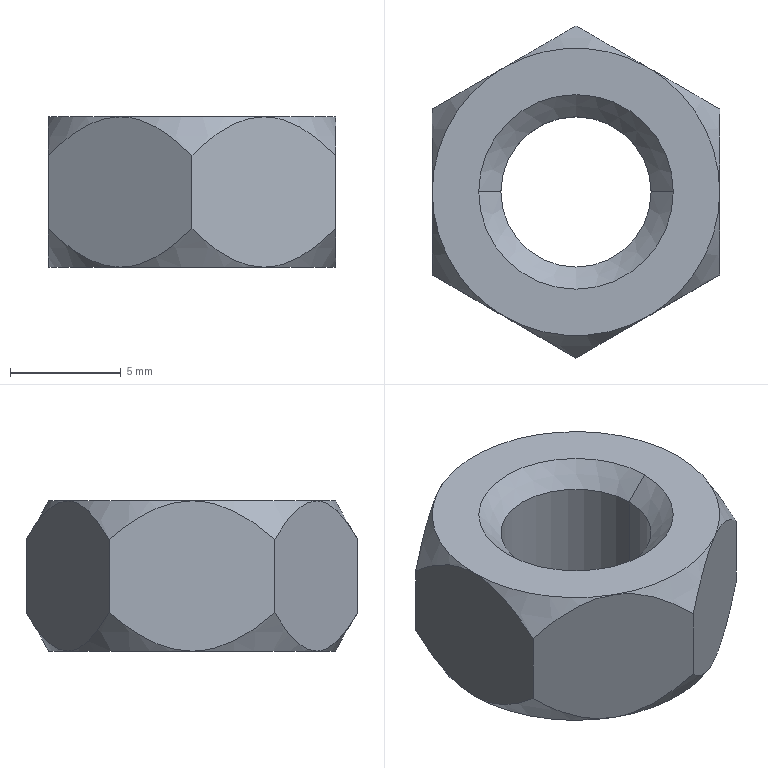Component | SolidWorks | Nut-3 | 1 solid | 26 faces | box 13 x 15.01 x 6.8 mm | volume 711 mm3 | cone 16 | plane 8 | cylinder 2 | commonest cylinder face diameters 6.8 x2
build123d program:
from build123d import *

# Parameters (mm, degrees)
BOSS_EXTRUDE1_DEPTH     = 3.4
SKETCH2_OUTSIDE_W       = 27.05
SKETCH2_OUTSIDE_H       = 29.062
SKETCH2_OUTSIDE_R       = 6.5
CUT_EXTRUDE1_DEPTH      = 6.8
CUT_EXTRUDE1_DRAFT      = -30
MIRROR1_COPY_1_SKETCH_W = 27.05
MIRROR1_COPY_1_SKETCH_H = 29.062
MIRROR1_COPY_1_SKETCH_R = 6.5
MIRROR1_COPY_1_DEPTH    = 6.8
MIRROR1_COPY_1_DRAFT    = -30
SKETCH5_W               = 3.4
SKETCH5_H               = 6.8
CHAMFER1_SIZE           = 1


with BuildPart() as part:
    # Sketch1 → Boss-Extrude1 (new, symmetric)
    with BuildSketch(Plane.XY):
        Polygon((0, 7.506), (-6.5, 3.753), (-6.5, -3.753), (0, -7.506), (6.5, -3.753), (6.5, 3.753), align=None)
    extrude(amount=BOSS_EXTRUDE1_DEPTH, both=True)


with BuildPart() as cut_extrude1_tool:
    # Sketch2 outside → Cut-Extrude1 (with draft: the straight prism first)
    with BuildSketch(Plane.XY.offset(3.4)):
        Rectangle(SKETCH2_OUTSIDE_W, SKETCH2_OUTSIDE_H)
        Circle(SKETCH2_OUTSIDE_R, mode=Mode.SUBTRACT)
    extrude(amount=-CUT_EXTRUDE1_DEPTH)
    # Cut-Extrude1: the draft: its side faces are tilted about the plane it starts from
    cut_extrude1_sides = [cut_extrude1_tool.faces().sort_by_distance(p)[0] for p in [
        (0, -14.531, 0),
        (13.525, 0, 0),
        (0, 14.531, 0),
        (-13.525, 0, 0),
        (-6.5, 0, 0),
    ]]
    draft(cut_extrude1_sides, Plane.XY.offset(3.4), CUT_EXTRUDE1_DRAFT)


with BuildPart() as part_1:
    add(part.part)

    # Cut-Extrude1: cut by cut_extrude1_tool
    add(cut_extrude1_tool.part, mode=Mode.SUBTRACT)


with BuildPart() as mirror1_copy_1_tool:
    # Mirror1 copy 1 sketch → Mirror1 copy 1 (with draft: the straight prism first)
    with BuildSketch(Plane(origin=(0, 0, -3.4), x_dir=(1, 0, 0), z_dir=(0, 0, -1))):
        Rectangle(MIRROR1_COPY_1_SKETCH_W, MIRROR1_COPY_1_SKETCH_H)
        Circle(MIRROR1_COPY_1_SKETCH_R, mode=Mode.SUBTRACT)
    extrude(amount=-MIRROR1_COPY_1_DEPTH)
    # Mirror1 copy 1: the draft: its side faces are tilted about the plane it starts from
    mirror1_copy_1_sides = [mirror1_copy_1_tool.faces().sort_by_distance(p)[0] for p in [
        (0, -14.531, 0),
        (13.525, 0, 0),
        (0, 14.531, 0),
        (-13.525, 0, 0),
        (-6.5, 0, 0),
    ]]
    draft(mirror1_copy_1_sides, Plane(origin=(0, 0, -3.4), x_dir=(1, 0, 0), z_dir=(0, 0, -1)), MIRROR1_COPY_1_DRAFT)


with BuildPart() as part_2:
    add(part_1.part)

    # Mirror1 copy 1: cut by mirror1_copy_1_tool
    add(mirror1_copy_1_tool.part, mode=Mode.SUBTRACT)

    # Sketch5 → M8 Tapped Hole1 (revolve, cut)
    with BuildSketch(Plane(origin=(0, 0, -3.4), x_dir=(0, 1, 0), z_dir=(1, 0, 0))):
        with Locations((1.7, 3.4)):
            Rectangle(SKETCH5_W, SKETCH5_H)
    revolve(axis=Axis((0, 0, -9.75), (0, 0, 1)), mode=Mode.SUBTRACT)

    # Chamfer1
    chamfer1_edges = [part_2.edges().sort_by_distance(p)[0] for p in [
        (0, -3.4, -3.4),
        (0, -3.4, 3.4),
    ]]
    chamfer(chamfer1_edges, length=CHAMFER1_SIZE)


solid = part_2.part

# Placed as in the assembly
solid = solid.moved(Location((-55.719, -28.485, 220.4), (0, 0, 0)))
STEP:
#1=CARTESIAN_POINT('',(-2.06,-1.121,8.583));
#2=VERTEX_POINT('',#1);
#3=CARTESIAN_POINT('',(-2.328,-1.121,8.583));
#4=VERTEX_POINT('',#3);
#5=CARTESIAN_POINT('',(-2.194,-1.121,8.583));
#6=DIRECTION('',(0.,0.,-1.));
#7=DIRECTION('',(-1.,0.,0.));
#8=AXIS2_PLACEMENT_3D('',#5,#6,#7);
#9=CIRCLE('',#8,0.1339);
#10=EDGE_CURVE('',#2,#4,#9,.T.);
#11=ORIENTED_EDGE('',*,*,#10,.F.);
#12=CARTESIAN_POINT('',(-2.02,-1.121,8.543));
#13=VERTEX_POINT('',#12);
#14=CARTESIAN_POINT('',(-2.02,-1.121,8.543));
#15=DIRECTION('',(0.7071,0.,-0.7071));
#16=VECTOR('',#15,39.37);
#17=LINE('',#14,#16);
#18=EDGE_CURVE('',#2,#13,#17,.T.);
#19=ORIENTED_EDGE('',*,*,#18,.T.);
#20=CARTESIAN_POINT('',(-2.367,-1.121,8.543));
#21=VERTEX_POINT('',#20);
#22=CARTESIAN_POINT('',(-2.194,-1.121,8.543));
#23=DIRECTION('',(0.,0.,1.));
#24=DIRECTION('',(-1.,0.,0.));
#25=AXIS2_PLACEMENT_3D('',#22,#23,#24);
#26=CIRCLE('',#25,0.1732);
#27=EDGE_CURVE('',#21,#13,#26,.T.);
#28=ORIENTED_EDGE('',*,*,#27,.F.);
#29=CARTESIAN_POINT('',(-2.367,-1.121,8.543));
#30=DIRECTION('',(-0.7071,0.,-0.7071));
#31=VECTOR('',#30,39.37);
#32=LINE('',#29,#31);
#33=EDGE_CURVE('',#4,#21,#32,.T.);
#34=ORIENTED_EDGE('',*,*,#33,.F.);
#35=EDGE_LOOP('',(#11,#19,#28,#34));
#36=FACE_OUTER_BOUND('',#35,.T.);
#37=CARTESIAN_POINT('',(-2.194,-1.121,8.543));
#38=DIRECTION('',(0.,0.,-1.));
#39=DIRECTION('',(-1.,0.,0.));
#40=AXIS2_PLACEMENT_3D('',#37,#38,#39);
#41=CONICAL_SURFACE('',#40,0.1732,0.7854);
#42=ADVANCED_FACE('',(#36),#41,.F.);
#43=CARTESIAN_POINT('',(-2.328,-1.121,8.772));
#44=VERTEX_POINT('',#43);
#45=CARTESIAN_POINT('',(-2.06,-1.121,8.772));
#46=VERTEX_POINT('',#45);
#47=CARTESIAN_POINT('',(-2.194,-1.121,8.772));
#48=DIRECTION('',(0.,0.,1.));
#49=DIRECTION('',(-1.,0.,0.));
#50=AXIS2_PLACEMENT_3D('',#47,#48,#49);
#51=CIRCLE('',#50,0.1339);
#52=EDGE_CURVE('',#44,#46,#51,.T.);
#53=ORIENTED_EDGE('',*,*,#52,.F.);
#54=CARTESIAN_POINT('',(-2.367,-1.121,8.811));
#55=VERTEX_POINT('',#54);
#56=CARTESIAN_POINT('',(-2.328,-1.121,8.772));
#57=DIRECTION('',(-0.7071,0.,0.7071));
#58=VECTOR('',#57,39.37);
#59=LINE('',#56,#58);
#60=EDGE_CURVE('',#44,#55,#59,.T.);
#61=ORIENTED_EDGE('',*,*,#60,.T.);
#62=CARTESIAN_POINT('',(-2.02,-1.121,8.811));
#63=VERTEX_POINT('',#62);
#64=CARTESIAN_POINT('',(-2.194,-1.121,8.811));
#65=DIRECTION('',(0.,0.,-1.));
#66=DIRECTION('',(-1.,0.,0.));
#67=AXIS2_PLACEMENT_3D('',#64,#65,#66);
#68=CIRCLE('',#67,0.1732);
#69=EDGE_CURVE('',#63,#55,#68,.T.);
#70=ORIENTED_EDGE('',*,*,#69,.F.);
#71=CARTESIAN_POINT('',(-2.06,-1.121,8.772));
#72=DIRECTION('',(0.7071,0.,0.7071));
#73=VECTOR('',#72,39.37);
#74=LINE('',#71,#73);
#75=EDGE_CURVE('',#46,#63,#74,.T.);
#76=ORIENTED_EDGE('',*,*,#75,.F.);
#77=EDGE_LOOP('',(#53,#61,#70,#76));
#78=FACE_OUTER_BOUND('',#77,.T.);
#79=CARTESIAN_POINT('',(-2.194,-1.121,8.772));
#80=DIRECTION('',(0.,0.,1.));
#81=DIRECTION('',(1.,0.,0.));
#82=AXIS2_PLACEMENT_3D('',#79,#80,#81);
#83=CONICAL_SURFACE('',#82,0.1339,0.7854);
#84=ADVANCED_FACE('',(#78),#83,.F.);
#85=ORIENTED_EDGE('',*,*,#10,.T.);
#86=CARTESIAN_POINT('',(-2.328,-1.121,8.811));
#87=DIRECTION('',(0.,0.,1.));
#88=VECTOR('',#87,39.37);
#89=LINE('',#86,#88);
#90=EDGE_CURVE('',#4,#44,#89,.T.);
#91=ORIENTED_EDGE('',*,*,#90,.T.);
#92=ORIENTED_EDGE('',*,*,#52,.T.);
#93=CARTESIAN_POINT('',(-2.06,-1.121,8.811));
#94=DIRECTION('',(0.,0.,1.));
#95=VECTOR('',#94,39.37);
#96=LINE('',#93,#95);
#97=EDGE_CURVE('',#2,#46,#96,.T.);
#98=ORIENTED_EDGE('',*,*,#97,.F.);
#99=EDGE_LOOP('',(#85,#91,#92,#98));
#100=FACE_OUTER_BOUND('',#99,.T.);
#101=CARTESIAN_POINT('',(-2.194,-1.121,8.811));
#102=DIRECTION('',(0.,0.,1.));
#103=DIRECTION('',(1.,0.,0.));
#104=AXIS2_PLACEMENT_3D('',#101,#102,#103);
#105=CYLINDRICAL_SURFACE('',#104,0.1339);
#106=ADVANCED_FACE('',(#100),#105,.F.);
#107=CARTESIAN_POINT('',(-2.45,-0.9737,8.612));
#108=VERTEX_POINT('',#107);
#109=CARTESIAN_POINT('',(-2.45,-0.9737,8.742));
#110=VERTEX_POINT('',#109);
#111=CARTESIAN_POINT('',(-2.45,-0.9737,8.543));
#112=DIRECTION('',(0.,0.,1.));
#113=VECTOR('',#112,39.37);
#114=LINE('',#111,#113);
#115=EDGE_CURVE('',#108,#110,#114,.T.);
#116=ORIENTED_EDGE('',*,*,#115,.T.);
#117=CARTESIAN_POINT('',(-2.322,-0.8998,8.811));
#118=VERTEX_POINT('',#117);
#119=CARTESIAN_POINT('',(-2.45,-0.9737,8.742));
#120=CARTESIAN_POINT('',(-2.44,-0.9685,8.752));
#121=CARTESIAN_POINT('',(-2.431,-0.9631,8.76));
#122=CARTESIAN_POINT('',(-2.412,-0.9518,8.776));
#123=CARTESIAN_POINT('',(-2.402,-0.946,8.784));
#124=CARTESIAN_POINT('',(-2.38,-0.9337,8.796));
#125=CARTESIAN_POINT('',(-2.369,-0.9271,8.802));
#126=CARTESIAN_POINT('',(-2.352,-0.9171,8.807));
#127=CARTESIAN_POINT('',(-2.346,-0.9137,8.809));
#128=CARTESIAN_POINT('',(-2.334,-0.9068,8.811));
#129=CARTESIAN_POINT('',(-2.328,-0.9033,8.811));
#130=CARTESIAN_POINT('',(-2.322,-0.8998,8.811));
#131=B_SPLINE_CURVE_WITH_KNOTS('',3,(#119,#120,#121,#122,#123,#124,#125,#126,#127,#128,#129,#130),.UNSPECIFIED.,.F.,.F.,(4,2,2,2,2,4),(0.0000003,0.001051,0.002101,0.003151,0.003676,0.004201),.UNSPECIFIED.);
#132=EDGE_CURVE('',#110,#118,#131,.T.);
#133=ORIENTED_EDGE('',*,*,#132,.T.);
#134=CARTESIAN_POINT('',(-2.194,-0.826,8.742));
#135=VERTEX_POINT('',#134);
#136=CARTESIAN_POINT('',(-2.322,-0.8998,8.811));
#137=CARTESIAN_POINT('',(-2.31,-0.8929,8.811));
#138=CARTESIAN_POINT('',(-2.298,-0.8861,8.809));
#139=CARTESIAN_POINT('',(-2.274,-0.8726,8.802));
#140=CARTESIAN_POINT('',(-2.263,-0.8662,8.796));
#141=CARTESIAN_POINT('',(-2.242,-0.8539,8.784));
#142=CARTESIAN_POINT('',(-2.232,-0.848,8.776));
#143=CARTESIAN_POINT('',(-2.212,-0.8367,8.76));
#144=CARTESIAN_POINT('',(-2.203,-0.8312,8.752));
#145=CARTESIAN_POINT('',(-2.194,-0.826,8.742));
#146=B_SPLINE_CURVE_WITH_KNOTS('',3,(#136,#137,#138,#139,#140,#141,#142,#143,#144,#145),.UNSPECIFIED.,.F.,.F.,(4,2,2,2,4),(0.004201,0.00525,0.006298,0.007347,0.008395),.UNSPECIFIED.);
#147=EDGE_CURVE('',#118,#135,#146,.T.);
#148=ORIENTED_EDGE('',*,*,#147,.T.);
#149=CARTESIAN_POINT('',(-2.194,-0.826,8.612));
#150=VERTEX_POINT('',#149);
#151=CARTESIAN_POINT('',(-2.194,-0.826,8.543));
#152=DIRECTION('',(0.,0.,1.));
#153=VECTOR('',#152,39.37);
#154=LINE('',#151,#153);
#155=EDGE_CURVE('',#150,#135,#154,.T.);
#156=ORIENTED_EDGE('',*,*,#155,.F.);
#157=CARTESIAN_POINT('',(-2.322,-0.8998,8.543));
#158=VERTEX_POINT('',#157);
#159=CARTESIAN_POINT('',(-2.322,-0.8998,8.543));
#160=CARTESIAN_POINT('',(-2.31,-0.8929,8.543));
#161=CARTESIAN_POINT('',(-2.298,-0.8861,8.545));
#162=CARTESIAN_POINT('',(-2.274,-0.8726,8.553));
#163=CARTESIAN_POINT('',(-2.263,-0.8662,8.558));
#164=CARTESIAN_POINT('',(-2.242,-0.8539,8.571));
#165=CARTESIAN_POINT('',(-2.232,-0.848,8.578));
#166=CARTESIAN_POINT('',(-2.212,-0.8367,8.594));
#167=CARTESIAN_POINT('',(-2.203,-0.8312,8.603));
#168=CARTESIAN_POINT('',(-2.194,-0.826,8.612));
#169=B_SPLINE_CURVE_WITH_KNOTS('',3,(#159,#160,#161,#162,#163,#164,#165,#166,#167,#168),.UNSPECIFIED.,.F.,.F.,(4,2,2,2,4),(0.004201,0.00525,0.006298,0.007347,0.008395),.UNSPECIFIED.);
#170=EDGE_CURVE('',#158,#150,#169,.T.);
#171=ORIENTED_EDGE('',*,*,#170,.F.);
#172=CARTESIAN_POINT('',(-2.45,-0.9737,8.612));
#173=CARTESIAN_POINT('',(-2.44,-0.9685,8.603));
#174=CARTESIAN_POINT('',(-2.431,-0.9631,8.594));
#175=CARTESIAN_POINT('',(-2.412,-0.9518,8.578));
#176=CARTESIAN_POINT('',(-2.402,-0.946,8.571));
#177=CARTESIAN_POINT('',(-2.38,-0.9337,8.558));
#178=CARTESIAN_POINT('',(-2.369,-0.9271,8.553));
#179=CARTESIAN_POINT('',(-2.352,-0.9171,8.547));
#180=CARTESIAN_POINT('',(-2.346,-0.9137,8.546));
#181=CARTESIAN_POINT('',(-2.334,-0.9068,8.544));
#182=CARTESIAN_POINT('',(-2.328,-0.9033,8.543));
#183=CARTESIAN_POINT('',(-2.322,-0.8998,8.543));
#184=B_SPLINE_CURVE_WITH_KNOTS('',3,(#172,#173,#174,#175,#176,#177,#178,#179,#180,#181,#182,#183),.UNSPECIFIED.,.F.,.F.,(4,2,2,2,2,4),(0.0000003,0.001051,0.002101,0.003151,0.003676,0.004201),.UNSPECIFIED.);
#185=EDGE_CURVE('',#108,#158,#184,.T.);
#186=ORIENTED_EDGE('',*,*,#185,.F.);
#187=EDGE_LOOP('',(#116,#133,#148,#156,#171,#186));
#188=FACE_OUTER_BOUND('',#187,.T.);
#189=CARTESIAN_POINT('',(-2.45,-0.9737,8.543));
#190=DIRECTION('',(0.5,-0.866,0.));
#191=DIRECTION('',(-0.866,-0.5,0.));
#192=AXIS2_PLACEMENT_3D('',#189,#190,#191);
#193=PLANE('',#192);
#194=ADVANCED_FACE('',(#188),#193,.F.);
#195=ORIENTED_EDGE('',*,*,#155,.T.);
#196=CARTESIAN_POINT('',(-2.066,-0.8998,8.811));
#197=VERTEX_POINT('',#196);
#198=CARTESIAN_POINT('',(-2.194,-0.826,8.742));
#199=CARTESIAN_POINT('',(-2.185,-0.8312,8.752));
#200=CARTESIAN_POINT('',(-2.175,-0.8366,8.76));
#201=CARTESIAN_POINT('',(-2.156,-0.8479,8.776));
#202=CARTESIAN_POINT('',(-2.146,-0.8537,8.784));
#203=CARTESIAN_POINT('',(-2.124,-0.866,8.796));
#204=CARTESIAN_POINT('',(-2.113,-0.8725,8.802));
#205=CARTESIAN_POINT('',(-2.096,-0.8826,8.807));
#206=CARTESIAN_POINT('',(-2.09,-0.886,8.809));
#207=CARTESIAN_POINT('',(-2.078,-0.8929,8.811));
#208=CARTESIAN_POINT('',(-2.072,-0.8964,8.811));
#209=CARTESIAN_POINT('',(-2.066,-0.8998,8.811));
#210=B_SPLINE_CURVE_WITH_KNOTS('',3,(#198,#199,#200,#201,#202,#203,#204,#205,#206,#207,#208,#209),.UNSPECIFIED.,.F.,.F.,(4,2,2,2,2,4),(0.0000003,0.001051,0.002101,0.003151,0.003676,0.004201),.UNSPECIFIED.);
#211=EDGE_CURVE('',#135,#197,#210,.T.);
#212=ORIENTED_EDGE('',*,*,#211,.T.);
#213=CARTESIAN_POINT('',(-1.938,-0.9737,8.742));
#214=VERTEX_POINT('',#213);
#215=CARTESIAN_POINT('',(-2.066,-0.8998,8.811));
#216=CARTESIAN_POINT('',(-2.054,-0.9068,8.811));
#217=CARTESIAN_POINT('',(-2.042,-0.9136,8.809));
#218=CARTESIAN_POINT('',(-2.019,-0.9271,8.802));
#219=CARTESIAN_POINT('',(-2.007,-0.9335,8.796));
#220=CARTESIAN_POINT('',(-1.986,-0.9458,8.784));
#221=CARTESIAN_POINT('',(-1.976,-0.9517,8.776));
#222=CARTESIAN_POINT('',(-1.956,-0.963,8.76));
#223=CARTESIAN_POINT('',(-1.947,-0.9685,8.752));
#224=CARTESIAN_POINT('',(-1.938,-0.9737,8.742));
#225=B_SPLINE_CURVE_WITH_KNOTS('',3,(#215,#216,#217,#218,#219,#220,#221,#222,#223,#224),.UNSPECIFIED.,.F.,.F.,(4,2,2,2,4),(0.004201,0.00525,0.006298,0.007347,0.008395),.UNSPECIFIED.);
#226=EDGE_CURVE('',#197,#214,#225,.T.);
#227=ORIENTED_EDGE('',*,*,#226,.T.);
#228=CARTESIAN_POINT('',(-1.938,-0.9737,8.612));
#229=VERTEX_POINT('',#228);
#230=CARTESIAN_POINT('',(-1.938,-0.9737,8.543));
#231=DIRECTION('',(0.,0.,1.));
#232=VECTOR('',#231,39.37);
#233=LINE('',#230,#232);
#234=EDGE_CURVE('',#229,#214,#233,.T.);
#235=ORIENTED_EDGE('',*,*,#234,.F.);
#236=CARTESIAN_POINT('',(-2.066,-0.8998,8.543));
#237=VERTEX_POINT('',#236);
#238=CARTESIAN_POINT('',(-2.066,-0.8998,8.543));
#239=CARTESIAN_POINT('',(-2.054,-0.9068,8.543));
#240=CARTESIAN_POINT('',(-2.042,-0.9136,8.545));
#241=CARTESIAN_POINT('',(-2.019,-0.9271,8.553));
#242=CARTESIAN_POINT('',(-2.007,-0.9335,8.558));
#243=CARTESIAN_POINT('',(-1.986,-0.9458,8.571));
#244=CARTESIAN_POINT('',(-1.976,-0.9517,8.578));
#245=CARTESIAN_POINT('',(-1.956,-0.963,8.594));
#246=CARTESIAN_POINT('',(-1.947,-0.9685,8.603));
#247=CARTESIAN_POINT('',(-1.938,-0.9737,8.612));
#248=B_SPLINE_CURVE_WITH_KNOTS('',3,(#238,#239,#240,#241,#242,#243,#244,#245,#246,#247),.UNSPECIFIED.,.F.,.F.,(4,2,2,2,4),(0.004201,0.00525,0.006298,0.007347,0.008395),.UNSPECIFIED.);
#249=EDGE_CURVE('',#237,#229,#248,.T.);
#250=ORIENTED_EDGE('',*,*,#249,.F.);
#251=CARTESIAN_POINT('',(-2.194,-0.826,8.612));
#252=CARTESIAN_POINT('',(-2.185,-0.8312,8.603));
#253=CARTESIAN_POINT('',(-2.175,-0.8366,8.594));
#254=CARTESIAN_POINT('',(-2.156,-0.8479,8.578));
#255=CARTESIAN_POINT('',(-2.146,-0.8537,8.571));
#256=CARTESIAN_POINT('',(-2.124,-0.866,8.558));
#257=CARTESIAN_POINT('',(-2.113,-0.8725,8.553));
#258=CARTESIAN_POINT('',(-2.096,-0.8826,8.547));
#259=CARTESIAN_POINT('',(-2.09,-0.886,8.546));
#260=CARTESIAN_POINT('',(-2.078,-0.8929,8.544));
#261=CARTESIAN_POINT('',(-2.072,-0.8964,8.543));
#262=CARTESIAN_POINT('',(-2.066,-0.8998,8.543));
#263=B_SPLINE_CURVE_WITH_KNOTS('',3,(#251,#252,#253,#254,#255,#256,#257,#258,#259,#260,#261,#262),.UNSPECIFIED.,.F.,.F.,(4,2,2,2,2,4),(0.0000003,0.001051,0.002101,0.003151,0.003676,0.004201),.UNSPECIFIED.);
#264=EDGE_CURVE('',#150,#237,#263,.T.);
#265=ORIENTED_EDGE('',*,*,#264,.F.);
#266=EDGE_LOOP('',(#195,#212,#227,#235,#250,#265));
#267=FACE_OUTER_BOUND('',#266,.T.);
#268=CARTESIAN_POINT('',(-2.194,-0.826,8.543));
#269=DIRECTION('',(-0.5,-0.866,0.));
#270=DIRECTION('',(-0.866,0.5,0.));
#271=AXIS2_PLACEMENT_3D('',#268,#269,#270);
#272=PLANE('',#271);
#273=ADVANCED_FACE('',(#267),#272,.F.);
#274=ORIENTED_EDGE('',*,*,#234,.T.);
#275=CARTESIAN_POINT('',(-1.938,-1.121,8.811));
#276=VERTEX_POINT('',#275);
#277=CARTESIAN_POINT('',(-1.938,-0.9737,8.742));
#278=CARTESIAN_POINT('',(-1.938,-0.9841,8.751));
#279=CARTESIAN_POINT('',(-1.938,-0.9948,8.76));
#280=CARTESIAN_POINT('',(-1.938,-1.017,8.776));
#281=CARTESIAN_POINT('',(-1.938,-1.029,8.783));
#282=CARTESIAN_POINT('',(-1.938,-1.053,8.796));
#283=CARTESIAN_POINT('',(-1.938,-1.067,8.802));
#284=CARTESIAN_POINT('',(-1.938,-1.087,8.807));
#285=CARTESIAN_POINT('',(-1.938,-1.094,8.809));
#286=CARTESIAN_POINT('',(-1.938,-1.107,8.811));
#287=CARTESIAN_POINT('',(-1.938,-1.114,8.811));
#288=CARTESIAN_POINT('',(-1.938,-1.121,8.811));
#289=B_SPLINE_CURVE_WITH_KNOTS('',3,(#277,#278,#279,#280,#281,#282,#283,#284,#285,#286,#287,#288),.UNSPECIFIED.,.F.,.F.,(4,2,2,2,2,4),(0.01696,0.01802,0.01907,0.02012,0.02065,0.02117),.UNSPECIFIED.);
#290=EDGE_CURVE('',#214,#276,#289,.T.);
#291=ORIENTED_EDGE('',*,*,#290,.T.);
#292=CARTESIAN_POINT('',(-1.938,-1.269,8.742));
#293=VERTEX_POINT('',#292);
#294=CARTESIAN_POINT('',(-1.938,-1.121,8.811));
#295=CARTESIAN_POINT('',(-1.938,-1.135,8.811));
#296=CARTESIAN_POINT('',(-1.938,-1.149,8.809));
#297=CARTESIAN_POINT('',(-1.938,-1.169,8.804));
#298=CARTESIAN_POINT('',(-1.938,-1.176,8.801));
#299=CARTESIAN_POINT('',(-1.938,-1.189,8.796));
#300=CARTESIAN_POINT('',(-1.938,-1.195,8.793));
#301=CARTESIAN_POINT('',(-1.938,-1.226,8.777));
#302=CARTESIAN_POINT('',(-1.938,-1.248,8.761));
#303=CARTESIAN_POINT('',(-1.938,-1.269,8.742));
#304=B_SPLINE_CURVE_WITH_KNOTS('',3,(#294,#295,#296,#297,#298,#299,#300,#301,#302,#303),.UNSPECIFIED.,.F.,.F.,(4,2,2,2,4),(0.02117,0.02222,0.02274,0.02326,0.02535),.UNSPECIFIED.);
#305=EDGE_CURVE('',#276,#293,#304,.T.);
#306=ORIENTED_EDGE('',*,*,#305,.T.);
#307=CARTESIAN_POINT('',(-1.938,-1.269,8.612));
#308=VERTEX_POINT('',#307);
#309=CARTESIAN_POINT('',(-1.938,-1.269,8.543));
#310=DIRECTION('',(0.,0.,1.));
#311=VECTOR('',#310,39.37);
#312=LINE('',#309,#311);
#313=EDGE_CURVE('',#308,#293,#312,.T.);
#314=ORIENTED_EDGE('',*,*,#313,.F.);
#315=CARTESIAN_POINT('',(-1.938,-1.121,8.543));
#316=VERTEX_POINT('',#315);
#317=CARTESIAN_POINT('',(-1.938,-1.121,8.543));
#318=CARTESIAN_POINT('',(-1.938,-1.135,8.543));
#319=CARTESIAN_POINT('',(-1.938,-1.149,8.545));
#320=CARTESIAN_POINT('',(-1.938,-1.169,8.551));
#321=CARTESIAN_POINT('',(-1.938,-1.176,8.553));
#322=CARTESIAN_POINT('',(-1.938,-1.189,8.558));
#323=CARTESIAN_POINT('',(-1.938,-1.195,8.561));
#324=CARTESIAN_POINT('',(-1.938,-1.226,8.577));
#325=CARTESIAN_POINT('',(-1.938,-1.248,8.594));
#326=CARTESIAN_POINT('',(-1.938,-1.269,8.612));
#327=B_SPLINE_CURVE_WITH_KNOTS('',3,(#317,#318,#319,#320,#321,#322,#323,#324,#325,#326),.UNSPECIFIED.,.F.,.F.,(4,2,2,2,4),(0.02117,0.02222,0.02274,0.02326,0.02535),.UNSPECIFIED.);
#328=EDGE_CURVE('',#316,#308,#327,.T.);
#329=ORIENTED_EDGE('',*,*,#328,.F.);
#330=CARTESIAN_POINT('',(-1.938,-0.9737,8.612));
#331=CARTESIAN_POINT('',(-1.938,-0.9841,8.603));
#332=CARTESIAN_POINT('',(-1.938,-0.9948,8.594));
#333=CARTESIAN_POINT('',(-1.938,-1.017,8.578));
#334=CARTESIAN_POINT('',(-1.938,-1.029,8.571));
#335=CARTESIAN_POINT('',(-1.938,-1.053,8.558));
#336=CARTESIAN_POINT('',(-1.938,-1.067,8.553));
#337=CARTESIAN_POINT('',(-1.938,-1.087,8.547));
#338=CARTESIAN_POINT('',(-1.938,-1.094,8.546));
#339=CARTESIAN_POINT('',(-1.938,-1.107,8.544));
#340=CARTESIAN_POINT('',(-1.938,-1.114,8.543));
#341=CARTESIAN_POINT('',(-1.938,-1.121,8.543));
#342=B_SPLINE_CURVE_WITH_KNOTS('',3,(#330,#331,#332,#333,#334,#335,#336,#337,#338,#339,#340,#341),.UNSPECIFIED.,.F.,.F.,(4,2,2,2,2,4),(0.01696,0.01802,0.01907,0.02012,0.02065,0.02117),.UNSPECIFIED.);
#343=EDGE_CURVE('',#229,#316,#342,.T.);
#344=ORIENTED_EDGE('',*,*,#343,.F.);
#345=EDGE_LOOP('',(#274,#291,#306,#314,#329,#344));
#346=FACE_OUTER_BOUND('',#345,.T.);
#347=CARTESIAN_POINT('',(-1.938,-0.9737,8.543));
#348=DIRECTION('',(-1.,0.,0.));
#349=DIRECTION('',(0.,1.,0.));
#350=AXIS2_PLACEMENT_3D('',#347,#348,#349);
#351=PLANE('',#350);
#352=ADVANCED_FACE('',(#346),#351,.F.);
#353=ORIENTED_EDGE('',*,*,#313,.T.);
#354=CARTESIAN_POINT('',(-2.066,-1.343,8.811));
#355=VERTEX_POINT('',#354);
#356=CARTESIAN_POINT('',(-1.938,-1.269,8.742));
#357=CARTESIAN_POINT('',(-1.947,-1.274,8.752));
#358=CARTESIAN_POINT('',(-1.956,-1.28,8.76));
#359=CARTESIAN_POINT('',(-1.976,-1.291,8.776));
#360=CARTESIAN_POINT('',(-1.986,-1.297,8.784));
#361=CARTESIAN_POINT('',(-2.007,-1.309,8.796));
#362=CARTESIAN_POINT('',(-2.018,-1.316,8.802));
#363=CARTESIAN_POINT('',(-2.036,-1.326,8.807));
#364=CARTESIAN_POINT('',(-2.042,-1.329,8.809));
#365=CARTESIAN_POINT('',(-2.054,-1.336,8.811));
#366=CARTESIAN_POINT('',(-2.06,-1.34,8.811));
#367=CARTESIAN_POINT('',(-2.066,-1.343,8.811));
#368=B_SPLINE_CURVE_WITH_KNOTS('',3,(#356,#357,#358,#359,#360,#361,#362,#363,#364,#365,#366,#367),.UNSPECIFIED.,.F.,.F.,(4,2,2,2,2,4),(0.0000003,0.001051,0.002101,0.003151,0.003676,0.004201),.UNSPECIFIED.);
#369=EDGE_CURVE('',#293,#355,#368,.T.);
#370=ORIENTED_EDGE('',*,*,#369,.T.);
#371=CARTESIAN_POINT('',(-2.194,-1.417,8.742));
#372=VERTEX_POINT('',#371);
#373=CARTESIAN_POINT('',(-2.066,-1.343,8.811));
#374=CARTESIAN_POINT('',(-2.078,-1.35,8.811));
#375=CARTESIAN_POINT('',(-2.09,-1.357,8.809));
#376=CARTESIAN_POINT('',(-2.113,-1.37,8.802));
#377=CARTESIAN_POINT('',(-2.124,-1.377,8.796));
#378=CARTESIAN_POINT('',(-2.145,-1.389,8.784));
#379=CARTESIAN_POINT('',(-2.155,-1.395,8.776));
#380=CARTESIAN_POINT('',(-2.175,-1.406,8.76));
#381=CARTESIAN_POINT('',(-2.185,-1.412,8.752));
#382=CARTESIAN_POINT('',(-2.194,-1.417,8.742));
#383=B_SPLINE_CURVE_WITH_KNOTS('',3,(#373,#374,#375,#376,#377,#378,#379,#380,#381,#382),.UNSPECIFIED.,.F.,.F.,(4,2,2,2,4),(0.004201,0.00525,0.006298,0.007347,0.008395),.UNSPECIFIED.);
#384=EDGE_CURVE('',#355,#372,#383,.T.);
#385=ORIENTED_EDGE('',*,*,#384,.T.);
#386=CARTESIAN_POINT('',(-2.194,-1.417,8.612));
#387=VERTEX_POINT('',#386);
#388=CARTESIAN_POINT('',(-2.194,-1.417,8.543));
#389=DIRECTION('',(0.,0.,1.));
#390=VECTOR('',#389,39.37);
#391=LINE('',#388,#390);
#392=EDGE_CURVE('',#387,#372,#391,.T.);
#393=ORIENTED_EDGE('',*,*,#392,.F.);
#394=CARTESIAN_POINT('',(-2.066,-1.343,8.543));
#395=VERTEX_POINT('',#394);
#396=CARTESIAN_POINT('',(-2.066,-1.343,8.543));
#397=CARTESIAN_POINT('',(-2.078,-1.35,8.543));
#398=CARTESIAN_POINT('',(-2.09,-1.357,8.545));
#399=CARTESIAN_POINT('',(-2.113,-1.37,8.553));
#400=CARTESIAN_POINT('',(-2.124,-1.377,8.558));
#401=CARTESIAN_POINT('',(-2.145,-1.389,8.571));
#402=CARTESIAN_POINT('',(-2.155,-1.395,8.578));
#403=CARTESIAN_POINT('',(-2.175,-1.406,8.594));
#404=CARTESIAN_POINT('',(-2.185,-1.412,8.603));
#405=CARTESIAN_POINT('',(-2.194,-1.417,8.612));
#406=B_SPLINE_CURVE_WITH_KNOTS('',3,(#396,#397,#398,#399,#400,#401,#402,#403,#404,#405),.UNSPECIFIED.,.F.,.F.,(4,2,2,2,4),(0.004201,0.00525,0.006298,0.007347,0.008395),.UNSPECIFIED.);
#407=EDGE_CURVE('',#395,#387,#406,.T.);
#408=ORIENTED_EDGE('',*,*,#407,.F.);
#409=CARTESIAN_POINT('',(-1.938,-1.269,8.612));
#410=CARTESIAN_POINT('',(-1.947,-1.274,8.603));
#411=CARTESIAN_POINT('',(-1.956,-1.28,8.594));
#412=CARTESIAN_POINT('',(-1.976,-1.291,8.578));
#413=CARTESIAN_POINT('',(-1.986,-1.297,8.571));
#414=CARTESIAN_POINT('',(-2.007,-1.309,8.558));
#415=CARTESIAN_POINT('',(-2.018,-1.316,8.553));
#416=CARTESIAN_POINT('',(-2.036,-1.326,8.547));
#417=CARTESIAN_POINT('',(-2.042,-1.329,8.546));
#418=CARTESIAN_POINT('',(-2.054,-1.336,8.544));
#419=CARTESIAN_POINT('',(-2.06,-1.34,8.543));
#420=CARTESIAN_POINT('',(-2.066,-1.343,8.543));
#421=B_SPLINE_CURVE_WITH_KNOTS('',3,(#409,#410,#411,#412,#413,#414,#415,#416,#417,#418,#419,#420),.UNSPECIFIED.,.F.,.F.,(4,2,2,2,2,4),(0.0000003,0.001051,0.002101,0.003151,0.003676,0.004201),.UNSPECIFIED.);
#422=EDGE_CURVE('',#308,#395,#421,.T.);
#423=ORIENTED_EDGE('',*,*,#422,.F.);
#424=EDGE_LOOP('',(#353,#370,#385,#393,#408,#423));
#425=FACE_OUTER_BOUND('',#424,.T.);
#426=CARTESIAN_POINT('',(-1.938,-1.269,8.543));
#427=DIRECTION('',(-0.5,0.866,0.));
#428=DIRECTION('',(0.866,0.5,0.));
#429=AXIS2_PLACEMENT_3D('',#426,#427,#428);
#430=PLANE('',#429);
#431=ADVANCED_FACE('',(#425),#430,.F.);
#432=ORIENTED_EDGE('',*,*,#392,.T.);
#433=CARTESIAN_POINT('',(-2.322,-1.343,8.811));
#434=VERTEX_POINT('',#433);
#435=CARTESIAN_POINT('',(-2.194,-1.417,8.742));
#436=CARTESIAN_POINT('',(-2.203,-1.412,8.752));
#437=CARTESIAN_POINT('',(-2.212,-1.406,8.76));
#438=CARTESIAN_POINT('',(-2.232,-1.395,8.776));
#439=CARTESIAN_POINT('',(-2.242,-1.389,8.784));
#440=CARTESIAN_POINT('',(-2.263,-1.377,8.796));
#441=CARTESIAN_POINT('',(-2.274,-1.37,8.802));
#442=CARTESIAN_POINT('',(-2.292,-1.36,8.807));
#443=CARTESIAN_POINT('',(-2.298,-1.357,8.809));
#444=CARTESIAN_POINT('',(-2.309,-1.35,8.811));
#445=CARTESIAN_POINT('',(-2.316,-1.347,8.811));
#446=CARTESIAN_POINT('',(-2.322,-1.343,8.811));
#447=B_SPLINE_CURVE_WITH_KNOTS('',3,(#435,#436,#437,#438,#439,#440,#441,#442,#443,#444,#445,#446),.UNSPECIFIED.,.F.,.F.,(4,2,2,2,2,4),(0.0000003,0.001051,0.002101,0.003151,0.003676,0.004201),.UNSPECIFIED.);
#448=EDGE_CURVE('',#372,#434,#447,.T.);
#449=ORIENTED_EDGE('',*,*,#448,.T.);
#450=CARTESIAN_POINT('',(-2.45,-1.269,8.742));
#451=VERTEX_POINT('',#450);
#452=CARTESIAN_POINT('',(-2.322,-1.343,8.811));
#453=CARTESIAN_POINT('',(-2.334,-1.336,8.811));
#454=CARTESIAN_POINT('',(-2.345,-1.329,8.809));
#455=CARTESIAN_POINT('',(-2.369,-1.316,8.802));
#456=CARTESIAN_POINT('',(-2.38,-1.309,8.796));
#457=CARTESIAN_POINT('',(-2.401,-1.297,8.784));
#458=CARTESIAN_POINT('',(-2.411,-1.291,8.776));
#459=CARTESIAN_POINT('',(-2.431,-1.28,8.76));
#460=CARTESIAN_POINT('',(-2.44,-1.274,8.752));
#461=CARTESIAN_POINT('',(-2.45,-1.269,8.742));
#462=B_SPLINE_CURVE_WITH_KNOTS('',3,(#452,#453,#454,#455,#456,#457,#458,#459,#460,#461),.UNSPECIFIED.,.F.,.F.,(4,2,2,2,4),(0.004201,0.00525,0.006298,0.007347,0.008395),.UNSPECIFIED.);
#463=EDGE_CURVE('',#434,#451,#462,.T.);
#464=ORIENTED_EDGE('',*,*,#463,.T.);
#465=CARTESIAN_POINT('',(-2.45,-1.269,8.612));
#466=VERTEX_POINT('',#465);
#467=CARTESIAN_POINT('',(-2.45,-1.269,8.543));
#468=DIRECTION('',(0.,0.,1.));
#469=VECTOR('',#468,39.37);
#470=LINE('',#467,#469);
#471=EDGE_CURVE('',#466,#451,#470,.T.);
#472=ORIENTED_EDGE('',*,*,#471,.F.);
#473=CARTESIAN_POINT('',(-2.322,-1.343,8.543));
#474=VERTEX_POINT('',#473);
#475=CARTESIAN_POINT('',(-2.322,-1.343,8.543));
#476=CARTESIAN_POINT('',(-2.334,-1.336,8.543));
#477=CARTESIAN_POINT('',(-2.345,-1.329,8.545));
#478=CARTESIAN_POINT('',(-2.369,-1.316,8.553));
#479=CARTESIAN_POINT('',(-2.38,-1.309,8.558));
#480=CARTESIAN_POINT('',(-2.401,-1.297,8.571));
#481=CARTESIAN_POINT('',(-2.411,-1.291,8.578));
#482=CARTESIAN_POINT('',(-2.431,-1.28,8.594));
#483=CARTESIAN_POINT('',(-2.44,-1.274,8.603));
#484=CARTESIAN_POINT('',(-2.45,-1.269,8.612));
#485=B_SPLINE_CURVE_WITH_KNOTS('',3,(#475,#476,#477,#478,#479,#480,#481,#482,#483,#484),.UNSPECIFIED.,.F.,.F.,(4,2,2,2,4),(0.004201,0.00525,0.006298,0.007347,0.008395),.UNSPECIFIED.);
#486=EDGE_CURVE('',#474,#466,#485,.T.);
#487=ORIENTED_EDGE('',*,*,#486,.F.);
#488=CARTESIAN_POINT('',(-2.194,-1.417,8.612));
#489=CARTESIAN_POINT('',(-2.203,-1.412,8.603));
#490=CARTESIAN_POINT('',(-2.212,-1.406,8.594));
#491=CARTESIAN_POINT('',(-2.232,-1.395,8.578));
#492=CARTESIAN_POINT('',(-2.242,-1.389,8.571));
#493=CARTESIAN_POINT('',(-2.263,-1.377,8.558));
#494=CARTESIAN_POINT('',(-2.274,-1.37,8.553));
#495=CARTESIAN_POINT('',(-2.292,-1.36,8.547));
#496=CARTESIAN_POINT('',(-2.298,-1.357,8.546));
#497=CARTESIAN_POINT('',(-2.309,-1.35,8.544));
#498=CARTESIAN_POINT('',(-2.316,-1.347,8.543));
#499=CARTESIAN_POINT('',(-2.322,-1.343,8.543));
#500=B_SPLINE_CURVE_WITH_KNOTS('',3,(#488,#489,#490,#491,#492,#493,#494,#495,#496,#497,#498,#499),.UNSPECIFIED.,.F.,.F.,(4,2,2,2,2,4),(0.0000003,0.001051,0.002101,0.003151,0.003676,0.004201),.UNSPECIFIED.);
#501=EDGE_CURVE('',#387,#474,#500,.T.);
#502=ORIENTED_EDGE('',*,*,#501,.F.);
#503=EDGE_LOOP('',(#432,#449,#464,#472,#487,#502));
#504=FACE_OUTER_BOUND('',#503,.T.);
#505=CARTESIAN_POINT('',(-2.194,-1.417,8.543));
#506=DIRECTION('',(0.5,0.866,0.));
#507=DIRECTION('',(0.866,-0.5,0.));
#508=AXIS2_PLACEMENT_3D('',#505,#506,#507);
#509=PLANE('',#508);
#510=ADVANCED_FACE('',(#504),#509,.F.);
#511=ORIENTED_EDGE('',*,*,#471,.T.);
#512=CARTESIAN_POINT('',(-2.45,-1.121,8.811));
#513=VERTEX_POINT('',#512);
#514=CARTESIAN_POINT('',(-2.45,-1.269,8.742));
#515=CARTESIAN_POINT('',(-2.45,-1.259,8.751));
#516=CARTESIAN_POINT('',(-2.45,-1.248,8.76));
#517=CARTESIAN_POINT('',(-2.45,-1.226,8.776));
#518=CARTESIAN_POINT('',(-2.45,-1.214,8.783));
#519=CARTESIAN_POINT('',(-2.45,-1.189,8.796));
#520=CARTESIAN_POINT('',(-2.45,-1.176,8.802));
#521=CARTESIAN_POINT('',(-2.45,-1.156,8.807));
#522=CARTESIAN_POINT('',(-2.45,-1.149,8.809));
#523=CARTESIAN_POINT('',(-2.45,-1.136,8.811));
#524=CARTESIAN_POINT('',(-2.45,-1.128,8.811));
#525=CARTESIAN_POINT('',(-2.45,-1.121,8.811));
#526=B_SPLINE_CURVE_WITH_KNOTS('',3,(#514,#515,#516,#517,#518,#519,#520,#521,#522,#523,#524,#525),.UNSPECIFIED.,.F.,.F.,(4,2,2,2,2,4),(0.01696,0.01802,0.01907,0.02012,0.02065,0.02117),.UNSPECIFIED.);
#527=EDGE_CURVE('',#451,#513,#526,.T.);
#528=ORIENTED_EDGE('',*,*,#527,.T.);
#529=CARTESIAN_POINT('',(-2.45,-1.121,8.811));
#530=CARTESIAN_POINT('',(-2.45,-1.108,8.811));
#531=CARTESIAN_POINT('',(-2.45,-1.094,8.809));
#532=CARTESIAN_POINT('',(-2.45,-1.074,8.804));
#533=CARTESIAN_POINT('',(-2.45,-1.067,8.801));
#534=CARTESIAN_POINT('',(-2.45,-1.054,8.796));
#535=CARTESIAN_POINT('',(-2.45,-1.048,8.793));
#536=CARTESIAN_POINT('',(-2.45,-1.017,8.777));
#537=CARTESIAN_POINT('',(-2.45,-0.9946,8.761));
#538=CARTESIAN_POINT('',(-2.45,-0.9737,8.742));
#539=B_SPLINE_CURVE_WITH_KNOTS('',3,(#529,#530,#531,#532,#533,#534,#535,#536,#537,#538),.UNSPECIFIED.,.F.,.F.,(4,2,2,2,4),(0.02117,0.02222,0.02274,0.02326,0.02535),.UNSPECIFIED.);
#540=EDGE_CURVE('',#513,#110,#539,.T.);
#541=ORIENTED_EDGE('',*,*,#540,.T.);
#542=ORIENTED_EDGE('',*,*,#115,.F.);
#543=CARTESIAN_POINT('',(-2.45,-1.121,8.543));
#544=VERTEX_POINT('',#543);
#545=CARTESIAN_POINT('',(-2.45,-1.121,8.543));
#546=CARTESIAN_POINT('',(-2.45,-1.108,8.543));
#547=CARTESIAN_POINT('',(-2.45,-1.094,8.545));
#548=CARTESIAN_POINT('',(-2.45,-1.074,8.551));
#549=CARTESIAN_POINT('',(-2.45,-1.067,8.553));
#550=CARTESIAN_POINT('',(-2.45,-1.054,8.558));
#551=CARTESIAN_POINT('',(-2.45,-1.048,8.561));
#552=CARTESIAN_POINT('',(-2.45,-1.017,8.577));
#553=CARTESIAN_POINT('',(-2.45,-0.9946,8.594));
#554=CARTESIAN_POINT('',(-2.45,-0.9737,8.612));
#555=B_SPLINE_CURVE_WITH_KNOTS('',3,(#545,#546,#547,#548,#549,#550,#551,#552,#553,#554),.UNSPECIFIED.,.F.,.F.,(4,2,2,2,4),(0.02117,0.02222,0.02274,0.02326,0.02535),.UNSPECIFIED.);
#556=EDGE_CURVE('',#544,#108,#555,.T.);
#557=ORIENTED_EDGE('',*,*,#556,.F.);
#558=CARTESIAN_POINT('',(-2.45,-1.269,8.612));
#559=CARTESIAN_POINT('',(-2.45,-1.259,8.603));
#560=CARTESIAN_POINT('',(-2.45,-1.248,8.594));
#561=CARTESIAN_POINT('',(-2.45,-1.226,8.578));
#562=CARTESIAN_POINT('',(-2.45,-1.214,8.571));
#563=CARTESIAN_POINT('',(-2.45,-1.189,8.558));
#564=CARTESIAN_POINT('',(-2.45,-1.176,8.553));
#565=CARTESIAN_POINT('',(-2.45,-1.156,8.547));
#566=CARTESIAN_POINT('',(-2.45,-1.149,8.546));
#567=CARTESIAN_POINT('',(-2.45,-1.136,8.544));
#568=CARTESIAN_POINT('',(-2.45,-1.128,8.543));
#569=CARTESIAN_POINT('',(-2.45,-1.121,8.543));
#570=B_SPLINE_CURVE_WITH_KNOTS('',3,(#558,#559,#560,#561,#562,#563,#564,#565,#566,#567,#568,#569),.UNSPECIFIED.,.F.,.F.,(4,2,2,2,2,4),(0.01696,0.01802,0.01907,0.02012,0.02065,0.02117),.UNSPECIFIED.);
#571=EDGE_CURVE('',#466,#544,#570,.T.);
#572=ORIENTED_EDGE('',*,*,#571,.F.);
#573=EDGE_LOOP('',(#511,#528,#541,#542,#557,#572));
#574=FACE_OUTER_BOUND('',#573,.T.);
#575=CARTESIAN_POINT('',(-2.45,-1.269,8.543));
#576=DIRECTION('',(1.,-0.,0.));
#577=DIRECTION('',(-0.,-1.,0.));
#578=AXIS2_PLACEMENT_3D('',#575,#576,#577);
#579=PLANE('',#578);
#580=ADVANCED_FACE('',(#574),#579,.F.);
#581=ORIENTED_EDGE('',*,*,#486,.T.);
#582=ORIENTED_EDGE('',*,*,#571,.T.);
#583=CARTESIAN_POINT('',(-2.194,-1.121,8.543));
#584=DIRECTION('',(0.,0.,-1.));
#585=DIRECTION('',(-1.,0.,0.));
#586=AXIS2_PLACEMENT_3D('',#583,#584,#585);
#587=CIRCLE('',#586,0.2559);
#588=EDGE_CURVE('',#474,#544,#587,.T.);
#589=ORIENTED_EDGE('',*,*,#588,.F.);
#590=EDGE_LOOP('',(#581,#582,#589));
#591=FACE_OUTER_BOUND('',#590,.T.);
#592=CARTESIAN_POINT('',(-2.194,-1.121,8.543));
#593=DIRECTION('',(0.,0.,1.));
#594=DIRECTION('',(-1.,0.,0.));
#595=AXIS2_PLACEMENT_3D('',#592,#593,#594);
#596=CONICAL_SURFACE('',#595,0.2559,0.5236);
#597=ADVANCED_FACE('',(#591),#596,.T.);
#598=ORIENTED_EDGE('',*,*,#407,.T.);
#599=ORIENTED_EDGE('',*,*,#501,.T.);
#600=CARTESIAN_POINT('',(-2.194,-1.121,8.543));
#601=DIRECTION('',(0.,0.,-1.));
#602=DIRECTION('',(-1.,0.,0.));
#603=AXIS2_PLACEMENT_3D('',#600,#601,#602);
#604=CIRCLE('',#603,0.2559);
#605=EDGE_CURVE('',#395,#474,#604,.T.);
#606=ORIENTED_EDGE('',*,*,#605,.F.);
#607=EDGE_LOOP('',(#598,#599,#606));
#608=FACE_OUTER_BOUND('',#607,.T.);
#609=CARTESIAN_POINT('',(-2.194,-1.121,8.543));
#610=DIRECTION('',(0.,0.,1.));
#611=DIRECTION('',(-1.,0.,0.));
#612=AXIS2_PLACEMENT_3D('',#609,#610,#611);
#613=CONICAL_SURFACE('',#612,0.2559,0.5236);
#614=ADVANCED_FACE('',(#608),#613,.T.);
#615=ORIENTED_EDGE('',*,*,#328,.T.);
#616=ORIENTED_EDGE('',*,*,#422,.T.);
#617=CARTESIAN_POINT('',(-2.194,-1.121,8.543));
#618=DIRECTION('',(0.,0.,-1.));
#619=DIRECTION('',(-1.,0.,0.));
#620=AXIS2_PLACEMENT_3D('',#617,#618,#619);
#621=CIRCLE('',#620,0.2559);
#622=EDGE_CURVE('',#316,#395,#621,.T.);
#623=ORIENTED_EDGE('',*,*,#622,.F.);
#624=EDGE_LOOP('',(#615,#616,#623));
#625=FACE_OUTER_BOUND('',#624,.T.);
#626=CARTESIAN_POINT('',(-2.194,-1.121,8.543));
#627=DIRECTION('',(0.,0.,1.));
#628=DIRECTION('',(-1.,0.,0.));
#629=AXIS2_PLACEMENT_3D('',#626,#627,#628);
#630=CONICAL_SURFACE('',#629,0.2559,0.5236);
#631=ADVANCED_FACE('',(#625),#630,.T.);
#632=ORIENTED_EDGE('',*,*,#249,.T.);
#633=ORIENTED_EDGE('',*,*,#343,.T.);
#634=CARTESIAN_POINT('',(-2.194,-1.121,8.543));
#635=DIRECTION('',(0.,0.,-1.));
#636=DIRECTION('',(-1.,0.,0.));
#637=AXIS2_PLACEMENT_3D('',#634,#635,#636);
#638=CIRCLE('',#637,0.2559);
#639=EDGE_CURVE('',#237,#316,#638,.T.);
#640=ORIENTED_EDGE('',*,*,#639,.F.);
#641=EDGE_LOOP('',(#632,#633,#640));
#642=FACE_OUTER_BOUND('',#641,.T.);
#643=CARTESIAN_POINT('',(-2.194,-1.121,8.543));
#644=DIRECTION('',(0.,0.,1.));
#645=DIRECTION('',(-1.,0.,0.));
#646=AXIS2_PLACEMENT_3D('',#643,#644,#645);
#647=CONICAL_SURFACE('',#646,0.2559,0.5236);
#648=ADVANCED_FACE('',(#642),#647,.T.);
#649=ORIENTED_EDGE('',*,*,#170,.T.);
#650=ORIENTED_EDGE('',*,*,#264,.T.);
#651=CARTESIAN_POINT('',(-2.194,-1.121,8.543));
#652=DIRECTION('',(0.,0.,-1.));
#653=DIRECTION('',(-1.,0.,0.));
#654=AXIS2_PLACEMENT_3D('',#651,#652,#653);
#655=CIRCLE('',#654,0.2559);
#656=EDGE_CURVE('',#158,#237,#655,.T.);
#657=ORIENTED_EDGE('',*,*,#656,.F.);
#658=EDGE_LOOP('',(#649,#650,#657));
#659=FACE_OUTER_BOUND('',#658,.T.);
#660=CARTESIAN_POINT('',(-2.194,-1.121,8.543));
#661=DIRECTION('',(0.,0.,1.));
#662=DIRECTION('',(-1.,0.,0.));
#663=AXIS2_PLACEMENT_3D('',#660,#661,#662);
#664=CONICAL_SURFACE('',#663,0.2559,0.5236);
#665=ADVANCED_FACE('',(#659),#664,.T.);
#666=ORIENTED_EDGE('',*,*,#185,.T.);
#667=CARTESIAN_POINT('',(-2.194,-1.121,8.543));
#668=DIRECTION('',(0.,0.,-1.));
#669=DIRECTION('',(-1.,0.,0.));
#670=AXIS2_PLACEMENT_3D('',#667,#668,#669);
#671=CIRCLE('',#670,0.2559);
#672=EDGE_CURVE('',#544,#158,#671,.T.);
#673=ORIENTED_EDGE('',*,*,#672,.F.);
#674=ORIENTED_EDGE('',*,*,#556,.T.);
#675=EDGE_LOOP('',(#666,#673,#674));
#676=FACE_OUTER_BOUND('',#675,.T.);
#677=CARTESIAN_POINT('',(-2.194,-1.121,8.543));
#678=DIRECTION('',(0.,0.,1.));
#679=DIRECTION('',(-1.,0.,0.));
#680=AXIS2_PLACEMENT_3D('',#677,#678,#679);
#681=CONICAL_SURFACE('',#680,0.2559,0.5236);
#682=ADVANCED_FACE('',(#676),#681,.T.);
#683=ORIENTED_EDGE('',*,*,#27,.T.);
#684=CARTESIAN_POINT('',(-2.194,-1.121,8.543));
#685=DIRECTION('',(0.,0.,1.));
#686=DIRECTION('',(-1.,0.,0.));
#687=AXIS2_PLACEMENT_3D('',#684,#685,#686);
#688=CIRCLE('',#687,0.1732);
#689=EDGE_CURVE('',#13,#21,#688,.T.);
#690=ORIENTED_EDGE('',*,*,#689,.T.);
#691=EDGE_LOOP('',(#683,#690));
#692=FACE_BOUND('',#691,.T.);
#693=ORIENTED_EDGE('',*,*,#588,.T.);
#694=ORIENTED_EDGE('',*,*,#672,.T.);
#695=ORIENTED_EDGE('',*,*,#656,.T.);
#696=ORIENTED_EDGE('',*,*,#639,.T.);
#697=ORIENTED_EDGE('',*,*,#622,.T.);
#698=ORIENTED_EDGE('',*,*,#605,.T.);
#699=EDGE_LOOP('',(#693,#694,#695,#696,#697,#698));
#700=FACE_OUTER_BOUND('',#699,.T.);
#701=CARTESIAN_POINT('',(-2.194,-1.121,8.543));
#702=DIRECTION('',(0.,0.,-1.));
#703=DIRECTION('',(-1.,0.,0.));
#704=AXIS2_PLACEMENT_3D('',#701,#702,#703);
#705=PLANE('',#704);
#706=ADVANCED_FACE('',(#692,#700),#705,.T.);
#707=ORIENTED_EDGE('',*,*,#540,.F.);
#708=CARTESIAN_POINT('',(-2.194,-1.121,8.811));
#709=DIRECTION('',(0.,0.,-1.));
#710=DIRECTION('',(-1.,0.,0.));
#711=AXIS2_PLACEMENT_3D('',#708,#709,#710);
#712=CIRCLE('',#711,0.2559);
#713=EDGE_CURVE('',#513,#118,#712,.T.);
#714=ORIENTED_EDGE('',*,*,#713,.T.);
#715=ORIENTED_EDGE('',*,*,#132,.F.);
#716=EDGE_LOOP('',(#707,#714,#715));
#717=FACE_OUTER_BOUND('',#716,.T.);
#718=CARTESIAN_POINT('',(-2.194,-1.121,8.811));
#719=DIRECTION('',(0.,0.,-1.));
#720=DIRECTION('',(-1.,0.,0.));
#721=AXIS2_PLACEMENT_3D('',#718,#719,#720);
#722=CONICAL_SURFACE('',#721,0.2559,0.5236);
#723=ADVANCED_FACE('',(#717),#722,.T.);
#724=CARTESIAN_POINT('',(-2.194,-1.121,8.811));
#725=DIRECTION('',(0.,0.,1.));
#726=DIRECTION('',(-1.,0.,0.));
#727=AXIS2_PLACEMENT_3D('',#724,#725,#726);
#728=CIRCLE('',#727,0.2559);
#729=EDGE_CURVE('',#197,#118,#728,.T.);
#730=ORIENTED_EDGE('',*,*,#729,.F.);
#731=ORIENTED_EDGE('',*,*,#211,.F.);
#732=ORIENTED_EDGE('',*,*,#147,.F.);
#733=EDGE_LOOP('',(#730,#731,#732));
#734=FACE_OUTER_BOUND('',#733,.T.);
#735=CARTESIAN_POINT('',(-2.194,-1.121,8.811));
#736=DIRECTION('',(0.,0.,-1.));
#737=DIRECTION('',(-1.,0.,0.));
#738=AXIS2_PLACEMENT_3D('',#735,#736,#737);
#739=CONICAL_SURFACE('',#738,0.2559,0.5236);
#740=ADVANCED_FACE('',(#734),#739,.T.);
#741=CARTESIAN_POINT('',(-2.194,-1.121,8.811));
#742=DIRECTION('',(0.,0.,1.));
#743=DIRECTION('',(-1.,0.,0.));
#744=AXIS2_PLACEMENT_3D('',#741,#742,#743);
#745=CIRCLE('',#744,0.2559);
#746=EDGE_CURVE('',#276,#197,#745,.T.);
#747=ORIENTED_EDGE('',*,*,#746,.F.);
#748=ORIENTED_EDGE('',*,*,#290,.F.);
#749=ORIENTED_EDGE('',*,*,#226,.F.);
#750=EDGE_LOOP('',(#747,#748,#749));
#751=FACE_OUTER_BOUND('',#750,.T.);
#752=CARTESIAN_POINT('',(-2.194,-1.121,8.811));
#753=DIRECTION('',(0.,0.,-1.));
#754=DIRECTION('',(-1.,0.,0.));
#755=AXIS2_PLACEMENT_3D('',#752,#753,#754);
#756=CONICAL_SURFACE('',#755,0.2559,0.5236);
#757=ADVANCED_FACE('',(#751),#756,.T.);
#758=CARTESIAN_POINT('',(-2.194,-1.121,8.811));
#759=DIRECTION('',(0.,0.,1.));
#760=DIRECTION('',(-1.,0.,0.));
#761=AXIS2_PLACEMENT_3D('',#758,#759,#760);
#762=CIRCLE('',#761,0.2559);
#763=EDGE_CURVE('',#355,#276,#762,.T.);
#764=ORIENTED_EDGE('',*,*,#763,.F.);
#765=ORIENTED_EDGE('',*,*,#369,.F.);
#766=ORIENTED_EDGE('',*,*,#305,.F.);
#767=EDGE_LOOP('',(#764,#765,#766));
#768=FACE_OUTER_BOUND('',#767,.T.);
#769=CARTESIAN_POINT('',(-2.194,-1.121,8.811));
#770=DIRECTION('',(0.,0.,-1.));
#771=DIRECTION('',(-1.,0.,0.));
#772=AXIS2_PLACEMENT_3D('',#769,#770,#771);
#773=CONICAL_SURFACE('',#772,0.2559,0.5236);
#774=ADVANCED_FACE('',(#768),#773,.T.);
#775=CARTESIAN_POINT('',(-2.194,-1.121,8.811));
#776=DIRECTION('',(0.,0.,1.));
#777=DIRECTION('',(-1.,0.,0.));
#778=AXIS2_PLACEMENT_3D('',#775,#776,#777);
#779=CIRCLE('',#778,0.2559);
#780=EDGE_CURVE('',#434,#355,#779,.T.);
#781=ORIENTED_EDGE('',*,*,#780,.F.);
#782=ORIENTED_EDGE('',*,*,#448,.F.);
#783=ORIENTED_EDGE('',*,*,#384,.F.);
#784=EDGE_LOOP('',(#781,#782,#783));
#785=FACE_OUTER_BOUND('',#784,.T.);
#786=CARTESIAN_POINT('',(-2.194,-1.121,8.811));
#787=DIRECTION('',(0.,0.,-1.));
#788=DIRECTION('',(-1.,0.,0.));
#789=AXIS2_PLACEMENT_3D('',#786,#787,#788);
#790=CONICAL_SURFACE('',#789,0.2559,0.5236);
#791=ADVANCED_FACE('',(#785),#790,.T.);
#792=CARTESIAN_POINT('',(-2.194,-1.121,8.811));
#793=DIRECTION('',(0.,0.,1.));
#794=DIRECTION('',(-1.,0.,0.));
#795=AXIS2_PLACEMENT_3D('',#792,#793,#794);
#796=CIRCLE('',#795,0.2559);
#797=EDGE_CURVE('',#513,#434,#796,.T.);
#798=ORIENTED_EDGE('',*,*,#797,.F.);
#799=ORIENTED_EDGE('',*,*,#527,.F.);
#800=ORIENTED_EDGE('',*,*,#463,.F.);
#801=EDGE_LOOP('',(#798,#799,#800));
#802=FACE_OUTER_BOUND('',#801,.T.);
#803=CARTESIAN_POINT('',(-2.194,-1.121,8.811));
#804=DIRECTION('',(0.,0.,-1.));
#805=DIRECTION('',(-1.,0.,0.));
#806=AXIS2_PLACEMENT_3D('',#803,#804,#805);
#807=CONICAL_SURFACE('',#806,0.2559,0.5236);
#808=ADVANCED_FACE('',(#802),#807,.T.);
#809=ORIENTED_EDGE('',*,*,#69,.T.);
#810=CARTESIAN_POINT('',(-2.194,-1.121,8.811));
#811=DIRECTION('',(0.,0.,-1.));
#812=DIRECTION('',(-1.,0.,0.));
#813=AXIS2_PLACEMENT_3D('',#810,#811,#812);
#814=CIRCLE('',#813,0.1732);
#815=EDGE_CURVE('',#55,#63,#814,.T.);
#816=ORIENTED_EDGE('',*,*,#815,.T.);
#817=EDGE_LOOP('',(#809,#816));
#818=FACE_BOUND('',#817,.T.);
#819=ORIENTED_EDGE('',*,*,#713,.F.);
#820=ORIENTED_EDGE('',*,*,#797,.T.);
#821=ORIENTED_EDGE('',*,*,#780,.T.);
#822=ORIENTED_EDGE('',*,*,#763,.T.);
#823=ORIENTED_EDGE('',*,*,#746,.T.);
#824=ORIENTED_EDGE('',*,*,#729,.T.);
#825=EDGE_LOOP('',(#819,#820,#821,#822,#823,#824));
#826=FACE_OUTER_BOUND('',#825,.T.);
#827=CARTESIAN_POINT('',(-2.194,-1.121,8.811));
#828=DIRECTION('',(0.,0.,-1.));
#829=DIRECTION('',(-1.,0.,0.));
#830=AXIS2_PLACEMENT_3D('',#827,#828,#829);
#831=PLANE('',#830);
#832=ADVANCED_FACE('',(#818,#826),#831,.F.);
#833=ORIENTED_EDGE('',*,*,#90,.F.);
#834=CARTESIAN_POINT('',(-2.194,-1.121,8.583));
#835=DIRECTION('',(0.,0.,-1.));
#836=DIRECTION('',(-1.,0.,0.));
#837=AXIS2_PLACEMENT_3D('',#834,#835,#836);
#838=CIRCLE('',#837,0.1339);
#839=EDGE_CURVE('',#4,#2,#838,.T.);
#840=ORIENTED_EDGE('',*,*,#839,.T.);
#841=ORIENTED_EDGE('',*,*,#97,.T.);
#842=CARTESIAN_POINT('',(-2.194,-1.121,8.772));
#843=DIRECTION('',(0.,0.,1.));
#844=DIRECTION('',(-1.,0.,0.));
#845=AXIS2_PLACEMENT_3D('',#842,#843,#844);
#846=CIRCLE('',#845,0.1339);
#847=EDGE_CURVE('',#46,#44,#846,.T.);
#848=ORIENTED_EDGE('',*,*,#847,.T.);
#849=EDGE_LOOP('',(#833,#840,#841,#848));
#850=FACE_OUTER_BOUND('',#849,.T.);
#851=CARTESIAN_POINT('',(-2.194,-1.121,8.811));
#852=DIRECTION('',(0.,0.,1.));
#853=DIRECTION('',(1.,0.,0.));
#854=AXIS2_PLACEMENT_3D('',#851,#852,#853);
#855=CYLINDRICAL_SURFACE('',#854,0.1339);
#856=ADVANCED_FACE('',(#850),#855,.F.);
#857=ORIENTED_EDGE('',*,*,#60,.F.);
#858=ORIENTED_EDGE('',*,*,#847,.F.);
#859=ORIENTED_EDGE('',*,*,#75,.T.);
#860=ORIENTED_EDGE('',*,*,#815,.F.);
#861=EDGE_LOOP('',(#857,#858,#859,#860));
#862=FACE_OUTER_BOUND('',#861,.T.);
#863=CARTESIAN_POINT('',(-2.194,-1.121,8.772));
#864=DIRECTION('',(0.,0.,1.));
#865=DIRECTION('',(1.,0.,0.));
#866=AXIS2_PLACEMENT_3D('',#863,#864,#865);
#867=CONICAL_SURFACE('',#866,0.1339,0.7854);
#868=ADVANCED_FACE('',(#862),#867,.F.);
#869=ORIENTED_EDGE('',*,*,#18,.F.);
#870=ORIENTED_EDGE('',*,*,#839,.F.);
#871=ORIENTED_EDGE('',*,*,#33,.T.);
#872=ORIENTED_EDGE('',*,*,#689,.F.);
#873=EDGE_LOOP('',(#869,#870,#871,#872));
#874=FACE_OUTER_BOUND('',#873,.T.);
#875=CARTESIAN_POINT('',(-2.194,-1.121,8.543));
#876=DIRECTION('',(0.,0.,-1.));
#877=DIRECTION('',(-1.,0.,0.));
#878=AXIS2_PLACEMENT_3D('',#875,#876,#877);
#879=CONICAL_SURFACE('',#878,0.1732,0.7854);
#880=ADVANCED_FACE('',(#874),#879,.F.);
#881=CLOSED_SHELL('',(#42,#84,#106,#194,#273,#352,#431,#510,#580,#597,#614,#631,#648,#665,#682,#706,#723,#740,#757,#774,#791,#808,#832,#856,#868,#880));
#882=MANIFOLD_SOLID_BREP('',#881);
#883=CARTESIAN_POINT('',(0.,0.,0.));
#884=DIRECTION('',(0.,0.,1.));
#885=DIRECTION('',(1.,0.,0.));
#886=AXIS2_PLACEMENT_3D('',#883,#884,#885);
#887=(LENGTH_UNIT()NAMED_UNIT(*)SI_UNIT($,.METRE.));
#888=LENGTH_MEASURE_WITH_UNIT(LENGTH_MEASURE(0.0254),#887);
#889=DIMENSIONAL_EXPONENTS(1.,0.,0.,0.,0.,0.,0.);
#890=(CONVERSION_BASED_UNIT('',#888)LENGTH_UNIT()NAMED_UNIT(#889));
#891=UNCERTAINTY_MEASURE_WITH_UNIT(LENGTH_MEASURE(0.00001),#890,'','');
#892=(NAMED_UNIT(*)PLANE_ANGLE_UNIT()SI_UNIT($,.RADIAN.));
#893=(NAMED_UNIT(*)SI_UNIT($,.STERADIAN.)SOLID_ANGLE_UNIT());
#894=(GEOMETRIC_REPRESENTATION_CONTEXT(3)GLOBAL_UNCERTAINTY_ASSIGNED_CONTEXT((#891))GLOBAL_UNIT_ASSIGNED_CONTEXT((#890,#892,#893))REPRESENTATION_CONTEXT('',''));
#895=ADVANCED_BREP_SHAPE_REPRESENTATION('',(#882,#886),#894);
#896=COLOUR_RGB('',0.7922,0.8196,0.9333);
#897=FILL_AREA_STYLE_COLOUR('',#896);
#898=FILL_AREA_STYLE('',(#897));
#899=SURFACE_STYLE_FILL_AREA(#898);
#900=SURFACE_SIDE_STYLE('',(#899));
#901=SURFACE_STYLE_USAGE(.BOTH.,#900);
#902=PRESENTATION_STYLE_ASSIGNMENT((#901));
#903=STYLED_ITEM('',(#902),#882);
#904=PRESENTATION_LAYER_ASSIGNMENT('','',(#903));
#905=(LENGTH_UNIT()NAMED_UNIT(*)SI_UNIT($,.METRE.));
#906=LENGTH_MEASURE_WITH_UNIT(LENGTH_MEASURE(0.0254),#905);
#907=DIMENSIONAL_EXPONENTS(1.,0.,0.,0.,0.,0.,0.);
#908=(CONVERSION_BASED_UNIT('',#906)LENGTH_UNIT()NAMED_UNIT(#907));
#909=UNCERTAINTY_MEASURE_WITH_UNIT(LENGTH_MEASURE(0.00001),#908,'','');
#910=(NAMED_UNIT(*)PLANE_ANGLE_UNIT()SI_UNIT($,.RADIAN.));
#911=(NAMED_UNIT(*)SI_UNIT($,.STERADIAN.)SOLID_ANGLE_UNIT());
#912=(GEOMETRIC_REPRESENTATION_CONTEXT(3)GLOBAL_UNCERTAINTY_ASSIGNED_CONTEXT((#909))GLOBAL_UNIT_ASSIGNED_CONTEXT((#908,#910,#911))REPRESENTATION_CONTEXT('',''));
#913=MECHANICAL_DESIGN_GEOMETRIC_PRESENTATION_REPRESENTATION('',(#903),#912);